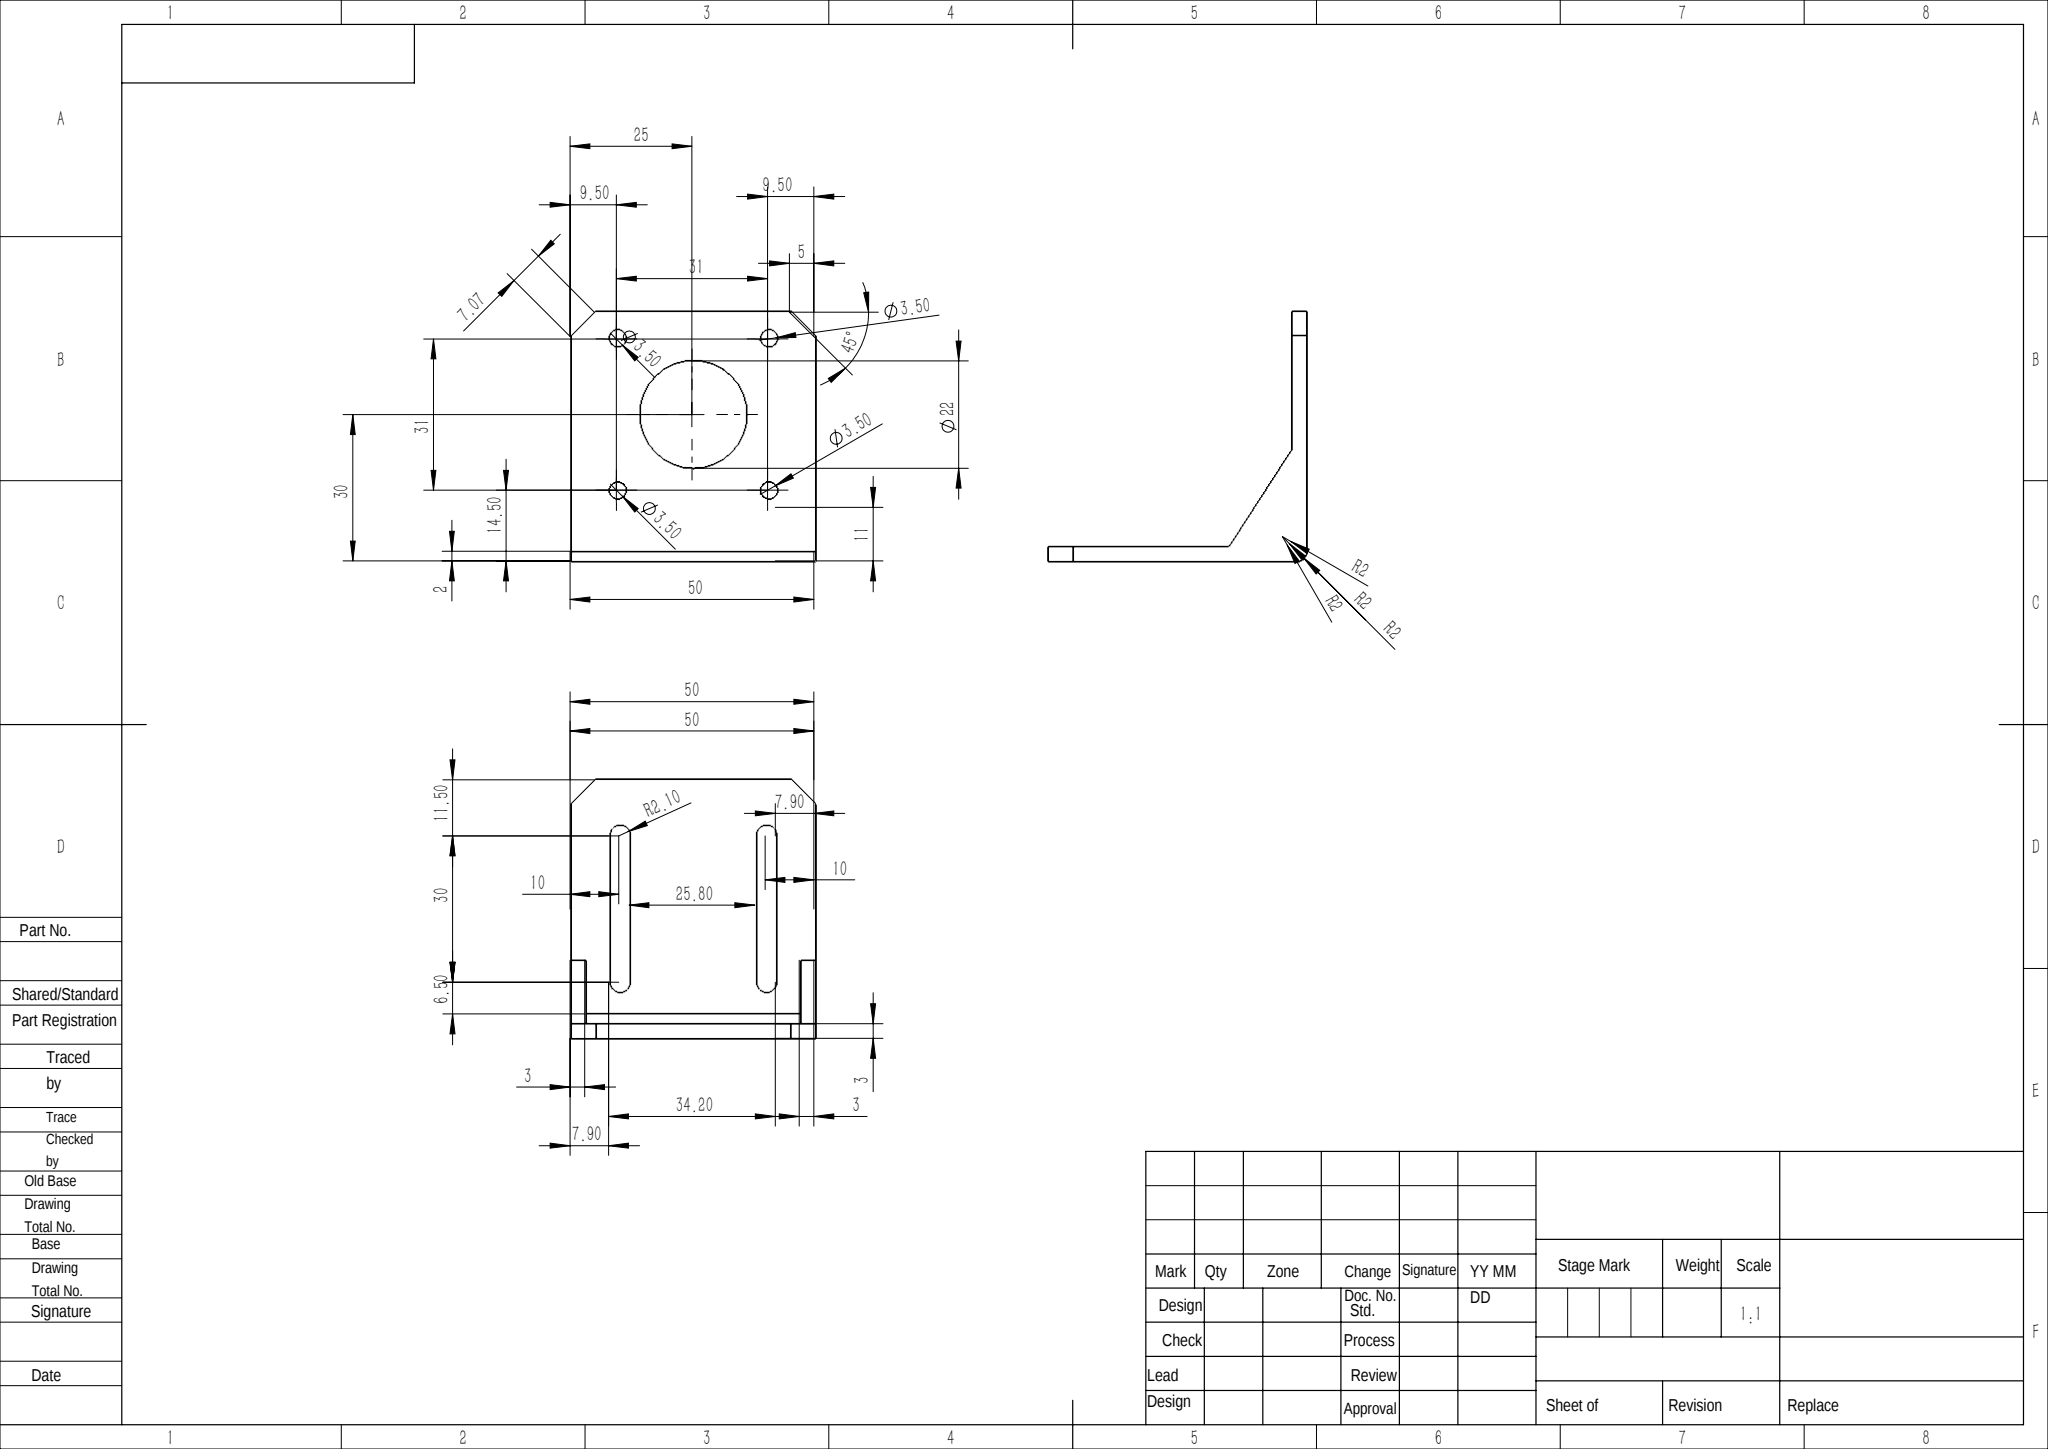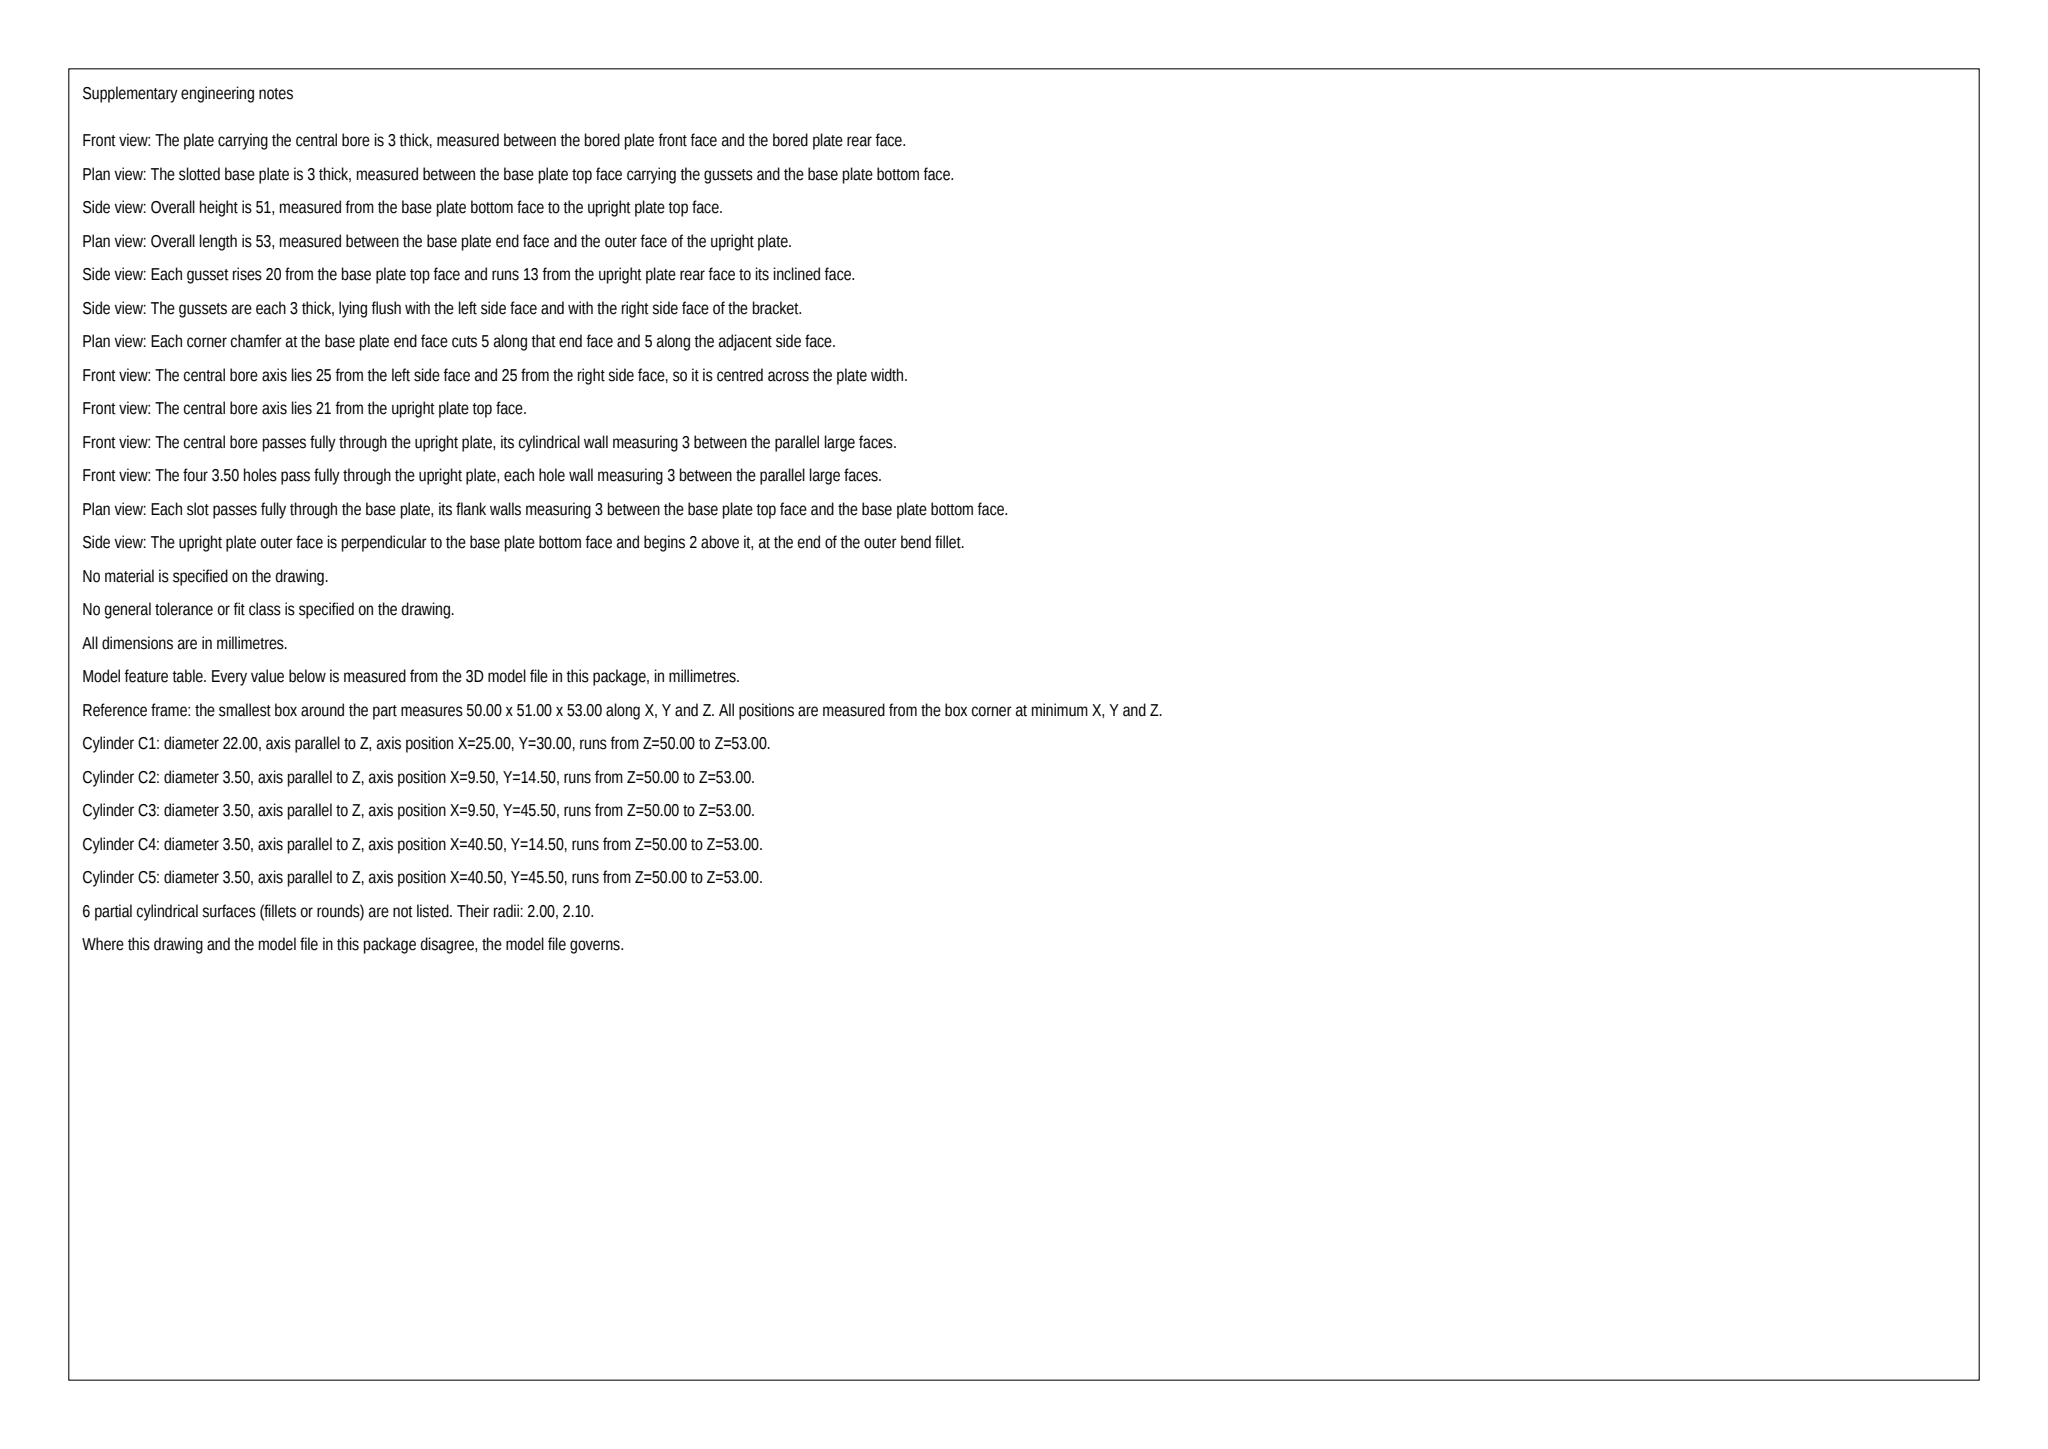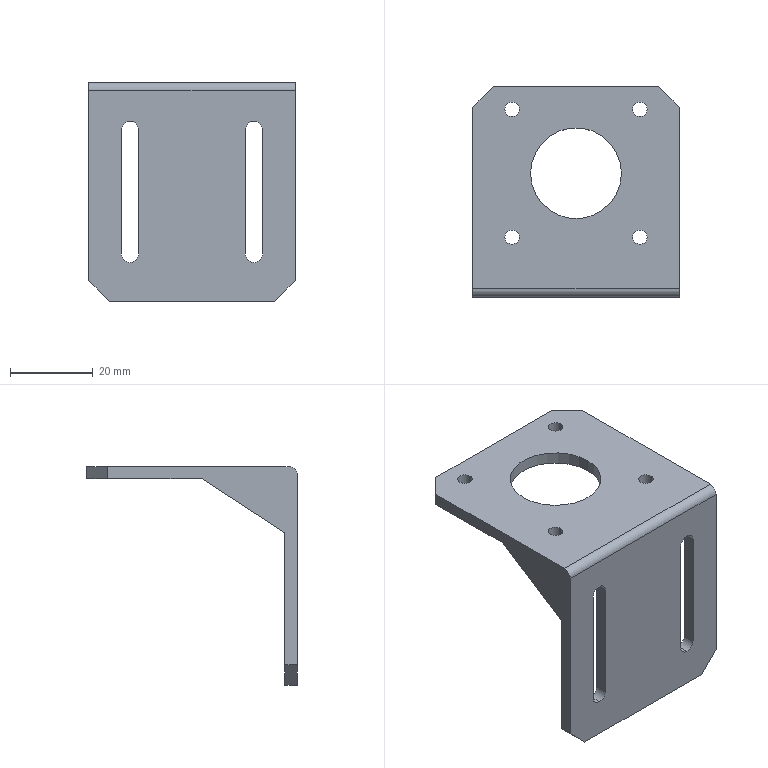Part | SolidWorks | mm | 1 solid | 38 faces | box 50 x 51 x 53 mm | volume 13680 mm3 | plane 20 | cylinder 18 | commonest cylinder face diameters 3.5 x8 4.2 x6 22 x2 4 x2
Drawing notes:
SIDE VIEW: VERT PLATE (WEB) THK 3 | from the solid: Planes normal to Y at y=0.0 (x 0-50, z 0-51) and y=3.0 (x 0-50, z 0-48) bound the upright leg: 3 mm thick
OVERALL DEPTH 51 (Y) FROM WEB OUTER FACE (Y=0) TO TOP PLATE REAR EDGE (Y=51) | from the solid: bbox_xyz = [50.0, 51.0, 53.0]; axis_plane y=0 (web outer face) and y=51 (rear face, x 5-45, z 50-53)
WEB (VERT PLATE) THK 3: 2X 5 X 45° CHAMFER AT CORNERS X=0-5 AND X=45-50, Z=0-5 | from the solid: inclined_planes angle [45,90,45], bbox_from [0,0,0] and [45,0,0], size [5,3,5]
2X GUSSET ANGLED EDGE 20 LONG IN Y, FROM Y=3 TO Y=23 (MEASURED FROM WEB OUTER FACE Y=0) | from the solid: inclined_planes angle [90,57,33], extent y 3 to 23, size [3,20,13]
2X GUSSET ANGLED EDGE 13 HIGH IN Z, FROM Z=37 TO Z=50 (TOP PLATE UNDERSIDE), PLATES AT X=0-3 AND X=47-50, THK 3 | from the solid: inclined_planes angle [90,57,33], bbox_from [0,3,37] and [47,3,37], size [3,20,13]; axis_plane z=50
build123d program:
from build123d import *

# Parameters (mm, degrees)
BOSS_EXTRUDE1_DEPTH = 50
BOSS_EXTRUDE2_DEPTH = 3
BOSS_EXTRUDE3_START = -3
BOSS_EXTRUDE3_DEPTH = 3
SKETCH5_R           = 11
SKETCH5_R_2         = 1.75
CUT_EXTRUDE1_DEPTH  = 3
CUT_EXTRUDE2_DEPTH  = 11
CHAMFER1_SIZE       = 5


with BuildPart() as part:
    # Sketch1 → Boss-Extrude1 (new body)
    with BuildSketch(Plane(origin=(0, 0, 0), x_dir=(0, 0, -1), z_dir=(1, 0, 0))):
        with BuildLine():
            Line((0, 2), (0, 51))
            Line((0, 51), (3, 51))
            Line((3, 51), (3, 5))
            ThreePointArc((3, 5), (3.586, 3.586), (5, 3))
            Line((5, 3), (53, 3))
            Line((53, 3), (53, 0))
            Line((53, 0), (2, 0))
            ThreePointArc((2, 0), (0.5858, 0.5858), (0, 2))
        make_face()
    extrude(amount=BOSS_EXTRUDE1_DEPTH)

    # Sketch3 → Boss-Extrude2 (add)
    with BuildSketch(Plane(origin=(0, 0, 0), x_dir=(0, 0, -1), z_dir=(1, 0, 0))):
        with BuildLine():
            Line((3, 5), (3, 23))
            Line((3, 23), (16, 3))
            Line((16, 3), (5, 3))
            ThreePointArc((5, 3), (3.586, 3.586), (3, 5))
        make_face()
    extrude(amount=BOSS_EXTRUDE2_DEPTH)

    # Sketch4 → Boss-Extrude3 (add)
    with BuildSketch(Plane(origin=(50, 0, 0), x_dir=(0, 0, -1), z_dir=(1, 0, 0)).offset(BOSS_EXTRUDE3_START)):
        with BuildLine():
            Line((3, 23), (3, 5))
            ThreePointArc((3, 5), (3.586, 3.586), (5, 3))
            Line((5, 3), (16, 3))
            Line((16, 3), (3, 23))
        make_face()
    extrude(amount=BOSS_EXTRUDE3_DEPTH)

    # Sketch5 → Cut-Extrude1 (cut)
    with BuildSketch(Plane.XY):
        with Locations((25, 30)):
            Circle(SKETCH5_R)
        with Locations((9.5, 45.5)):
            Circle(SKETCH5_R_2)
        with Locations((40.5, 45.5)):
            Circle(SKETCH5_R_2)
        with Locations((9.5, 14.5)):
            Circle(SKETCH5_R_2)
        with Locations((40.5, 14.5)):
            Circle(SKETCH5_R_2)
    extrude(amount=-CUT_EXTRUDE1_DEPTH, mode=Mode.SUBTRACT)

    # Sketch6 → Cut-Extrude2 (cut)
    with BuildSketch(Plane(origin=(0, 0, 0), x_dir=(1, 0, 0), z_dir=(0, 1, 0))):
        with BuildLine():
            Line((7.9, 41.5), (7.9, 11.5))
            ThreePointArc((7.9, 11.5), (10, 9.4), (12.1, 11.5))
            Line((12.1, 11.5), (12.1, 41.5))
            ThreePointArc((12.1, 41.5), (10, 43.6), (7.9, 41.5))
        make_face()
        with BuildLine():
            Line((37.9, 41.5), (37.9, 11.5))
            ThreePointArc((37.9, 11.5), (40, 9.4), (42.1, 11.5))
            Line((42.1, 11.5), (42.1, 41.5))
            ThreePointArc((42.1, 41.5), (40, 43.6), (37.9, 41.5))
        make_face()
    extrude(amount=CUT_EXTRUDE2_DEPTH, mode=Mode.SUBTRACT)

    # Chamfer1
    chamfer1_edges = [part.edges().sort_by_distance(p)[0] for p in [
        (0, 51, -1.5),
        (50, 1.5, -53),
        (50, 51, -1.5),
        (0, 1.5, -53),
    ]]
    chamfer(chamfer1_edges, length=CHAMFER1_SIZE)


solid = part.part